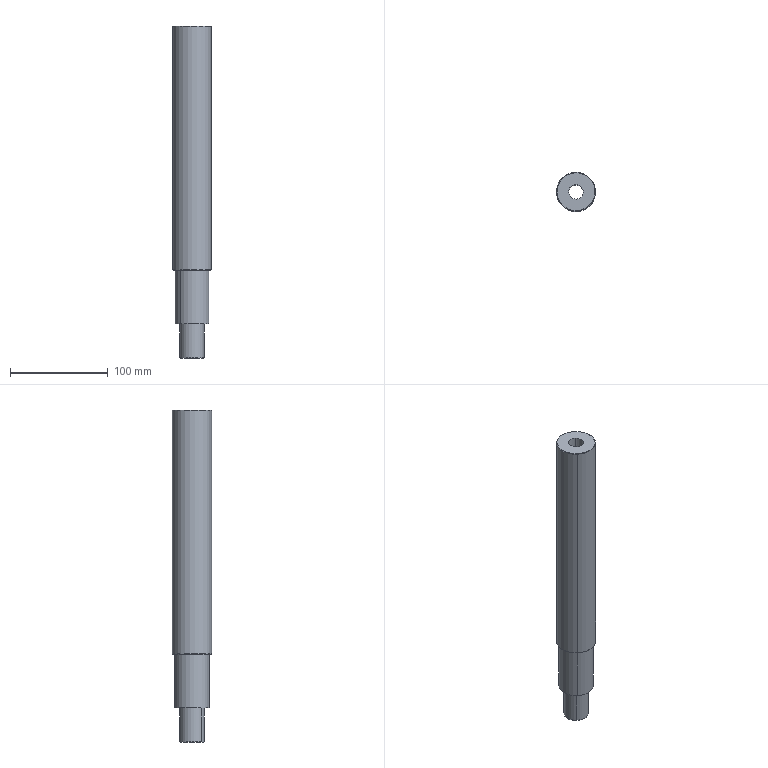Component | SolidWorks | 8TC-A17001-20-02HangingShaft-1 | 1 solid | 18 faces | box 40 x 40 x 340 mm | volume 324132 mm3 | cylinder 8 | cone 6 | plane 4 | commonest cylinder face diameters 40 x2 35 x2 25 x2 15 x2 | material #45
build123d program:
from build123d import *

# Parameters (mm, degrees)
CHAMFER1_SIZE = 0.5


with BuildPart() as part:
    # Sketch1 → Revolve1 (revolve)
    with BuildSketch(Plane(origin=(0, 0, 0), x_dir=(1, 0, 0), z_dir=(0, 1, 0)), mode=Mode.PRIVATE) as revolve1_sk:
        Polygon((0, 7.5), (0, 12.5), (35, 12.5), (35, 17.5), (90, 17.5), (90, 20), (340, 20), (340, 7.5), align=None)
    revolve(revolve1_sk.sketch.rotate(Axis((0, 0, 0), (1, 0, 0)), 180), axis=Axis((0, 0, 0), (1, 0, 0)))

    # Chamfer1
    chamfer1_edges = [part.edges().sort_by_distance(p)[0] for p in [
        (340, 0, -20),
        (90, 0, -20),
        (0, 0, -12.5),
    ]]
    chamfer(chamfer1_edges, length=CHAMFER1_SIZE)


solid = part.part

# Placed as in the assembly
solid = solid.moved(Location((733.029, 200.722, -47.5), (0, -90, 0)))
STEP:
#1=COLOUR_RGB('',0.7922,0.8196,0.9333);
#2=FILL_AREA_STYLE_COLOUR('',#1);
#3=FILL_AREA_STYLE('',(#2));
#4=SURFACE_STYLE_FILL_AREA(#3);
#5=SURFACE_SIDE_STYLE('',(#4));
#6=SURFACE_STYLE_USAGE(.BOTH.,#5);
#7=PRESENTATION_STYLE_ASSIGNMENT((#6));
#8=CARTESIAN_POINT('',(28.356,7.322,11.516));
#9=VERTEX_POINT('',#8);
#10=CARTESIAN_POINT('',(29.362,8.482,11.516));
#11=VERTEX_POINT('',#10);
#12=CARTESIAN_POINT('',(28.859,7.902,11.516));
#13=DIRECTION('',(0.,0.,1.));
#14=DIRECTION('',(0.6551,0.7555,0.));
#15=AXIS2_PLACEMENT_3D('',#12,#13,#14);
#16=CIRCLE('',#15,0.7677);
#17=EDGE_CURVE('',#9,#11,#16,.T.);
#18=ORIENTED_EDGE('',*,*,#17,.F.);
#19=CARTESIAN_POINT('',(28.344,7.308,11.496));
#20=VERTEX_POINT('',#19);
#21=CARTESIAN_POINT('',(28.344,7.308,11.496));
#22=DIRECTION('',(-0.4632,-0.5342,-0.7071));
#23=VECTOR('',#22,39.37);
#24=LINE('',#21,#23);
#25=EDGE_CURVE('',#9,#20,#24,.T.);
#26=ORIENTED_EDGE('',*,*,#25,.T.);
#27=CARTESIAN_POINT('',(29.375,8.497,11.496));
#28=VERTEX_POINT('',#27);
#29=CARTESIAN_POINT('',(28.859,7.902,11.496));
#30=DIRECTION('',(-0.,-0.,-1.));
#31=DIRECTION('',(0.6551,0.7555,0.));
#32=AXIS2_PLACEMENT_3D('',#29,#30,#31);
#33=CIRCLE('',#32,0.7874);
#34=EDGE_CURVE('',#28,#20,#33,.T.);
#35=ORIENTED_EDGE('',*,*,#34,.F.);
#36=CARTESIAN_POINT('',(29.375,8.497,11.496));
#37=DIRECTION('',(0.4632,0.5342,-0.7071));
#38=VECTOR('',#37,39.37);
#39=LINE('',#36,#38);
#40=EDGE_CURVE('',#11,#28,#39,.T.);
#41=ORIENTED_EDGE('',*,*,#40,.F.);
#42=EDGE_LOOP('',(#18,#26,#35,#41));
#43=FACE_OUTER_BOUND('',#42,.T.);
#44=CARTESIAN_POINT('',(28.859,7.902,11.496));
#45=DIRECTION('',(-0.,-0.,-1.));
#46=DIRECTION('',(0.6551,0.7555,0.));
#47=AXIS2_PLACEMENT_3D('',#44,#45,#46);
#48=CONICAL_SURFACE('',#47,0.7874,0.7854);
#49=ADVANCED_FACE('',(#43),#48,.T.);
#50=CARTESIAN_POINT('',(29.169,8.259,-1.87));
#51=VERTEX_POINT('',#50);
#52=CARTESIAN_POINT('',(28.55,7.545,-1.87));
#53=VERTEX_POINT('',#52);
#54=CARTESIAN_POINT('',(28.859,7.902,-1.87));
#55=DIRECTION('',(-0.,-0.,-1.));
#56=DIRECTION('',(-0.6551,-0.7555,0.));
#57=AXIS2_PLACEMENT_3D('',#54,#55,#56);
#58=CIRCLE('',#57,0.4724);
#59=EDGE_CURVE('',#51,#53,#58,.T.);
#60=ORIENTED_EDGE('',*,*,#59,.F.);
#61=CARTESIAN_POINT('',(29.182,8.274,-1.85));
#62=VERTEX_POINT('',#61);
#63=CARTESIAN_POINT('',(29.169,8.259,-1.87));
#64=DIRECTION('',(0.4632,0.5342,0.7071));
#65=VECTOR('',#64,39.37);
#66=LINE('',#63,#65);
#67=EDGE_CURVE('',#51,#62,#66,.T.);
#68=ORIENTED_EDGE('',*,*,#67,.T.);
#69=CARTESIAN_POINT('',(28.537,7.531,-1.85));
#70=VERTEX_POINT('',#69);
#71=CARTESIAN_POINT('',(28.859,7.902,-1.85));
#72=DIRECTION('',(0.,0.,1.));
#73=DIRECTION('',(-0.6551,-0.7555,0.));
#74=AXIS2_PLACEMENT_3D('',#71,#72,#73);
#75=CIRCLE('',#74,0.4921);
#76=EDGE_CURVE('',#70,#62,#75,.T.);
#77=ORIENTED_EDGE('',*,*,#76,.F.);
#78=CARTESIAN_POINT('',(28.55,7.545,-1.87));
#79=DIRECTION('',(-0.4632,-0.5342,0.7071));
#80=VECTOR('',#79,39.37);
#81=LINE('',#78,#80);
#82=EDGE_CURVE('',#53,#70,#81,.T.);
#83=ORIENTED_EDGE('',*,*,#82,.F.);
#84=EDGE_LOOP('',(#60,#68,#77,#83));
#85=FACE_OUTER_BOUND('',#84,.T.);
#86=CARTESIAN_POINT('',(28.859,7.902,-1.87));
#87=DIRECTION('',(0.,0.,1.));
#88=DIRECTION('',(-0.6551,-0.7555,0.));
#89=AXIS2_PLACEMENT_3D('',#86,#87,#88);
#90=CONICAL_SURFACE('',#89,0.4724,0.7854);
#91=ADVANCED_FACE('',(#85),#90,.T.);
#92=CARTESIAN_POINT('',(29.362,8.482,1.673));
#93=VERTEX_POINT('',#92);
#94=CARTESIAN_POINT('',(28.356,7.322,1.673));
#95=VERTEX_POINT('',#94);
#96=CARTESIAN_POINT('',(28.859,7.902,1.673));
#97=DIRECTION('',(-0.,-0.,-1.));
#98=DIRECTION('',(-0.6551,-0.7555,0.));
#99=AXIS2_PLACEMENT_3D('',#96,#97,#98);
#100=CIRCLE('',#99,0.7677);
#101=EDGE_CURVE('',#93,#95,#100,.T.);
#102=ORIENTED_EDGE('',*,*,#101,.F.);
#103=CARTESIAN_POINT('',(29.375,8.497,1.693));
#104=VERTEX_POINT('',#103);
#105=CARTESIAN_POINT('',(29.362,8.482,1.673));
#106=DIRECTION('',(0.4632,0.5342,0.7071));
#107=VECTOR('',#106,39.37);
#108=LINE('',#105,#107);
#109=EDGE_CURVE('',#93,#104,#108,.T.);
#110=ORIENTED_EDGE('',*,*,#109,.T.);
#111=CARTESIAN_POINT('',(28.344,7.308,1.693));
#112=VERTEX_POINT('',#111);
#113=CARTESIAN_POINT('',(28.859,7.902,1.693));
#114=DIRECTION('',(0.,0.,1.));
#115=DIRECTION('',(-0.6551,-0.7555,0.));
#116=AXIS2_PLACEMENT_3D('',#113,#114,#115);
#117=CIRCLE('',#116,0.7874);
#118=EDGE_CURVE('',#112,#104,#117,.T.);
#119=ORIENTED_EDGE('',*,*,#118,.F.);
#120=CARTESIAN_POINT('',(28.356,7.322,1.673));
#121=DIRECTION('',(-0.4632,-0.5342,0.7071));
#122=VECTOR('',#121,39.37);
#123=LINE('',#120,#122);
#124=EDGE_CURVE('',#95,#112,#123,.T.);
#125=ORIENTED_EDGE('',*,*,#124,.F.);
#126=EDGE_LOOP('',(#102,#110,#119,#125));
#127=FACE_OUTER_BOUND('',#126,.T.);
#128=CARTESIAN_POINT('',(28.859,7.902,1.673));
#129=DIRECTION('',(0.,0.,1.));
#130=DIRECTION('',(-0.6551,-0.7555,0.));
#131=AXIS2_PLACEMENT_3D('',#128,#129,#130);
#132=CONICAL_SURFACE('',#131,0.7677,0.7854);
#133=ADVANCED_FACE('',(#127),#132,.T.);
#134=ORIENTED_EDGE('',*,*,#34,.T.);
#135=CARTESIAN_POINT('',(28.344,7.308,-1.87));
#136=DIRECTION('',(-0.,-0.,-1.));
#137=VECTOR('',#136,39.37);
#138=LINE('',#135,#137);
#139=EDGE_CURVE('',#20,#112,#138,.T.);
#140=ORIENTED_EDGE('',*,*,#139,.T.);
#141=ORIENTED_EDGE('',*,*,#118,.T.);
#142=CARTESIAN_POINT('',(29.375,8.497,-1.87));
#143=DIRECTION('',(-0.,-0.,-1.));
#144=VECTOR('',#143,39.37);
#145=LINE('',#142,#144);
#146=EDGE_CURVE('',#28,#104,#145,.T.);
#147=ORIENTED_EDGE('',*,*,#146,.F.);
#148=EDGE_LOOP('',(#134,#140,#141,#147));
#149=FACE_OUTER_BOUND('',#148,.T.);
#150=CARTESIAN_POINT('',(28.859,7.902,-1.87));
#151=DIRECTION('',(-0.,-0.,-1.));
#152=DIRECTION('',(0.6551,0.7555,0.));
#153=AXIS2_PLACEMENT_3D('',#150,#151,#152);
#154=CYLINDRICAL_SURFACE('',#153,0.7874);
#155=ADVANCED_FACE('',(#149),#154,.T.);
#156=CARTESIAN_POINT('',(29.311,8.423,1.673));
#157=VERTEX_POINT('',#156);
#158=CARTESIAN_POINT('',(28.408,7.382,1.673));
#159=VERTEX_POINT('',#158);
#160=CARTESIAN_POINT('',(28.859,7.902,1.673));
#161=DIRECTION('',(-0.,-0.,-1.));
#162=DIRECTION('',(0.6551,0.7555,0.));
#163=AXIS2_PLACEMENT_3D('',#160,#161,#162);
#164=CIRCLE('',#163,0.689);
#165=EDGE_CURVE('',#157,#159,#164,.T.);
#166=ORIENTED_EDGE('',*,*,#165,.T.);
#167=CARTESIAN_POINT('',(28.408,7.382,-0.4921));
#168=VERTEX_POINT('',#167);
#169=CARTESIAN_POINT('',(28.408,7.382,-1.87));
#170=DIRECTION('',(-0.,-0.,-1.));
#171=VECTOR('',#170,39.37);
#172=LINE('',#169,#171);
#173=EDGE_CURVE('',#159,#168,#172,.T.);
#174=ORIENTED_EDGE('',*,*,#173,.T.);
#175=CARTESIAN_POINT('',(29.311,8.423,-0.4921));
#176=VERTEX_POINT('',#175);
#177=CARTESIAN_POINT('',(28.859,7.902,-0.4921));
#178=DIRECTION('',(-0.,-0.,-1.));
#179=DIRECTION('',(0.6551,0.7555,0.));
#180=AXIS2_PLACEMENT_3D('',#177,#178,#179);
#181=CIRCLE('',#180,0.689);
#182=EDGE_CURVE('',#176,#168,#181,.T.);
#183=ORIENTED_EDGE('',*,*,#182,.F.);
#184=CARTESIAN_POINT('',(29.311,8.423,-1.87));
#185=DIRECTION('',(-0.,-0.,-1.));
#186=VECTOR('',#185,39.37);
#187=LINE('',#184,#186);
#188=EDGE_CURVE('',#157,#176,#187,.T.);
#189=ORIENTED_EDGE('',*,*,#188,.F.);
#190=EDGE_LOOP('',(#166,#174,#183,#189));
#191=FACE_OUTER_BOUND('',#190,.T.);
#192=CARTESIAN_POINT('',(28.859,7.902,-1.87));
#193=DIRECTION('',(-0.,-0.,-1.));
#194=DIRECTION('',(0.6551,0.7555,0.));
#195=AXIS2_PLACEMENT_3D('',#192,#193,#194);
#196=CYLINDRICAL_SURFACE('',#195,0.689);
#197=ADVANCED_FACE('',(#191),#196,.T.);
#198=CARTESIAN_POINT('',(29.182,8.274,-0.4921));
#199=VERTEX_POINT('',#198);
#200=CARTESIAN_POINT('',(28.537,7.531,-0.4921));
#201=VERTEX_POINT('',#200);
#202=CARTESIAN_POINT('',(28.859,7.902,-0.4921));
#203=DIRECTION('',(-0.,-0.,-1.));
#204=DIRECTION('',(0.6551,0.7555,0.));
#205=AXIS2_PLACEMENT_3D('',#202,#203,#204);
#206=CIRCLE('',#205,0.4921);
#207=EDGE_CURVE('',#199,#201,#206,.T.);
#208=ORIENTED_EDGE('',*,*,#207,.T.);
#209=CARTESIAN_POINT('',(28.537,7.531,-1.87));
#210=DIRECTION('',(-0.,-0.,-1.));
#211=VECTOR('',#210,39.37);
#212=LINE('',#209,#211);
#213=EDGE_CURVE('',#201,#70,#212,.T.);
#214=ORIENTED_EDGE('',*,*,#213,.T.);
#215=ORIENTED_EDGE('',*,*,#76,.T.);
#216=CARTESIAN_POINT('',(29.182,8.274,-1.87));
#217=DIRECTION('',(-0.,-0.,-1.));
#218=VECTOR('',#217,39.37);
#219=LINE('',#216,#218);
#220=EDGE_CURVE('',#199,#62,#219,.T.);
#221=ORIENTED_EDGE('',*,*,#220,.F.);
#222=EDGE_LOOP('',(#208,#214,#215,#221));
#223=FACE_OUTER_BOUND('',#222,.T.);
#224=CARTESIAN_POINT('',(28.859,7.902,-1.87));
#225=DIRECTION('',(-0.,-0.,-1.));
#226=DIRECTION('',(0.6551,0.7555,0.));
#227=AXIS2_PLACEMENT_3D('',#224,#225,#226);
#228=CYLINDRICAL_SURFACE('',#227,0.4921);
#229=ADVANCED_FACE('',(#223),#228,.T.);
#230=CARTESIAN_POINT('',(28.666,7.679,11.516));
#231=VERTEX_POINT('',#230);
#232=CARTESIAN_POINT('',(29.053,8.126,11.516));
#233=VERTEX_POINT('',#232);
#234=CARTESIAN_POINT('',(28.859,7.902,11.516));
#235=DIRECTION('',(-0.,-0.,-1.));
#236=DIRECTION('',(0.6551,0.7555,0.));
#237=AXIS2_PLACEMENT_3D('',#234,#235,#236);
#238=CIRCLE('',#237,0.2953);
#239=EDGE_CURVE('',#231,#233,#238,.T.);
#240=ORIENTED_EDGE('',*,*,#239,.F.);
#241=CARTESIAN_POINT('',(28.666,7.679,-1.87));
#242=VERTEX_POINT('',#241);
#243=CARTESIAN_POINT('',(28.666,7.679,-1.87));
#244=DIRECTION('',(-0.,-0.,-1.));
#245=VECTOR('',#244,39.37);
#246=LINE('',#243,#245);
#247=EDGE_CURVE('',#231,#242,#246,.T.);
#248=ORIENTED_EDGE('',*,*,#247,.T.);
#249=CARTESIAN_POINT('',(29.053,8.126,-1.87));
#250=VERTEX_POINT('',#249);
#251=CARTESIAN_POINT('',(28.859,7.902,-1.87));
#252=DIRECTION('',(-0.,-0.,-1.));
#253=DIRECTION('',(0.6551,0.7555,0.));
#254=AXIS2_PLACEMENT_3D('',#251,#252,#253);
#255=CIRCLE('',#254,0.2953);
#256=EDGE_CURVE('',#242,#250,#255,.T.);
#257=ORIENTED_EDGE('',*,*,#256,.T.);
#258=CARTESIAN_POINT('',(29.053,8.126,-1.87));
#259=DIRECTION('',(-0.,-0.,-1.));
#260=VECTOR('',#259,39.37);
#261=LINE('',#258,#260);
#262=EDGE_CURVE('',#233,#250,#261,.T.);
#263=ORIENTED_EDGE('',*,*,#262,.F.);
#264=EDGE_LOOP('',(#240,#248,#257,#263));
#265=FACE_OUTER_BOUND('',#264,.T.);
#266=CARTESIAN_POINT('',(28.859,7.902,-1.87));
#267=DIRECTION('',(-0.,-0.,-1.));
#268=DIRECTION('',(0.6551,0.7555,0.));
#269=AXIS2_PLACEMENT_3D('',#266,#267,#268);
#270=CYLINDRICAL_SURFACE('',#269,0.2953);
#271=ADVANCED_FACE('',(#265),#270,.F.);
#272=ORIENTED_EDGE('',*,*,#247,.F.);
#273=CARTESIAN_POINT('',(28.859,7.902,11.516));
#274=DIRECTION('',(-0.,-0.,-1.));
#275=DIRECTION('',(0.6551,0.7555,0.));
#276=AXIS2_PLACEMENT_3D('',#273,#274,#275);
#277=CIRCLE('',#276,0.2953);
#278=EDGE_CURVE('',#233,#231,#277,.T.);
#279=ORIENTED_EDGE('',*,*,#278,.F.);
#280=ORIENTED_EDGE('',*,*,#262,.T.);
#281=CARTESIAN_POINT('',(28.859,7.902,-1.87));
#282=DIRECTION('',(-0.,-0.,-1.));
#283=DIRECTION('',(0.6551,0.7555,0.));
#284=AXIS2_PLACEMENT_3D('',#281,#282,#283);
#285=CIRCLE('',#284,0.2953);
#286=EDGE_CURVE('',#250,#242,#285,.T.);
#287=ORIENTED_EDGE('',*,*,#286,.T.);
#288=EDGE_LOOP('',(#272,#279,#280,#287));
#289=FACE_OUTER_BOUND('',#288,.T.);
#290=CARTESIAN_POINT('',(28.859,7.902,-1.87));
#291=DIRECTION('',(-0.,-0.,-1.));
#292=DIRECTION('',(0.6551,0.7555,0.));
#293=AXIS2_PLACEMENT_3D('',#290,#291,#292);
#294=CYLINDRICAL_SURFACE('',#293,0.2953);
#295=ADVANCED_FACE('',(#289),#294,.F.);
#296=CARTESIAN_POINT('',(28.859,7.902,-1.87));
#297=DIRECTION('',(-0.,-0.,-1.));
#298=DIRECTION('',(-0.6551,-0.7555,0.));
#299=AXIS2_PLACEMENT_3D('',#296,#297,#298);
#300=CIRCLE('',#299,0.4724);
#301=EDGE_CURVE('',#53,#51,#300,.T.);
#302=ORIENTED_EDGE('',*,*,#301,.T.);
#303=ORIENTED_EDGE('',*,*,#59,.T.);
#304=EDGE_LOOP('',(#302,#303));
#305=FACE_OUTER_BOUND('',#304,.T.);
#306=ORIENTED_EDGE('',*,*,#286,.F.);
#307=ORIENTED_EDGE('',*,*,#256,.F.);
#308=EDGE_LOOP('',(#306,#307));
#309=FACE_BOUND('',#308,.T.);
#310=CARTESIAN_POINT('',(28.666,7.679,-1.87));
#311=DIRECTION('',(0.,0.,1.));
#312=DIRECTION('',(-0.6551,-0.7555,0.));
#313=AXIS2_PLACEMENT_3D('',#310,#311,#312);
#314=PLANE('',#313);
#315=ADVANCED_FACE('',(#305,#309),#314,.F.);
#316=ORIENTED_EDGE('',*,*,#213,.F.);
#317=CARTESIAN_POINT('',(28.859,7.902,-0.4921));
#318=DIRECTION('',(-0.,-0.,-1.));
#319=DIRECTION('',(0.6551,0.7555,0.));
#320=AXIS2_PLACEMENT_3D('',#317,#318,#319);
#321=CIRCLE('',#320,0.4921);
#322=EDGE_CURVE('',#201,#199,#321,.T.);
#323=ORIENTED_EDGE('',*,*,#322,.T.);
#324=ORIENTED_EDGE('',*,*,#220,.T.);
#325=CARTESIAN_POINT('',(28.859,7.902,-1.85));
#326=DIRECTION('',(0.,0.,1.));
#327=DIRECTION('',(-0.6551,-0.7555,0.));
#328=AXIS2_PLACEMENT_3D('',#325,#326,#327);
#329=CIRCLE('',#328,0.4921);
#330=EDGE_CURVE('',#62,#70,#329,.T.);
#331=ORIENTED_EDGE('',*,*,#330,.T.);
#332=EDGE_LOOP('',(#316,#323,#324,#331));
#333=FACE_OUTER_BOUND('',#332,.T.);
#334=CARTESIAN_POINT('',(28.859,7.902,-1.87));
#335=DIRECTION('',(-0.,-0.,-1.));
#336=DIRECTION('',(0.6551,0.7555,0.));
#337=AXIS2_PLACEMENT_3D('',#334,#335,#336);
#338=CYLINDRICAL_SURFACE('',#337,0.4921);
#339=ADVANCED_FACE('',(#333),#338,.T.);
#340=ORIENTED_EDGE('',*,*,#207,.F.);
#341=ORIENTED_EDGE('',*,*,#322,.F.);
#342=EDGE_LOOP('',(#340,#341));
#343=FACE_BOUND('',#342,.T.);
#344=ORIENTED_EDGE('',*,*,#182,.T.);
#345=CARTESIAN_POINT('',(28.859,7.902,-0.4921));
#346=DIRECTION('',(-0.,-0.,-1.));
#347=DIRECTION('',(0.6551,0.7555,0.));
#348=AXIS2_PLACEMENT_3D('',#345,#346,#347);
#349=CIRCLE('',#348,0.689);
#350=EDGE_CURVE('',#168,#176,#349,.T.);
#351=ORIENTED_EDGE('',*,*,#350,.T.);
#352=EDGE_LOOP('',(#344,#351));
#353=FACE_OUTER_BOUND('',#352,.T.);
#354=CARTESIAN_POINT('',(28.537,7.531,-0.4921));
#355=DIRECTION('',(0.,0.,1.));
#356=DIRECTION('',(-0.6551,-0.7555,0.));
#357=AXIS2_PLACEMENT_3D('',#354,#355,#356);
#358=PLANE('',#357);
#359=ADVANCED_FACE('',(#343,#353),#358,.F.);
#360=ORIENTED_EDGE('',*,*,#173,.F.);
#361=CARTESIAN_POINT('',(28.859,7.902,1.673));
#362=DIRECTION('',(-0.,-0.,-1.));
#363=DIRECTION('',(0.6551,0.7555,0.));
#364=AXIS2_PLACEMENT_3D('',#361,#362,#363);
#365=CIRCLE('',#364,0.689);
#366=EDGE_CURVE('',#159,#157,#365,.T.);
#367=ORIENTED_EDGE('',*,*,#366,.T.);
#368=ORIENTED_EDGE('',*,*,#188,.T.);
#369=ORIENTED_EDGE('',*,*,#350,.F.);
#370=EDGE_LOOP('',(#360,#367,#368,#369));
#371=FACE_OUTER_BOUND('',#370,.T.);
#372=CARTESIAN_POINT('',(28.859,7.902,-1.87));
#373=DIRECTION('',(-0.,-0.,-1.));
#374=DIRECTION('',(0.6551,0.7555,0.));
#375=AXIS2_PLACEMENT_3D('',#372,#373,#374);
#376=CYLINDRICAL_SURFACE('',#375,0.689);
#377=ADVANCED_FACE('',(#371),#376,.T.);
#378=CARTESIAN_POINT('',(28.859,7.902,1.673));
#379=DIRECTION('',(-0.,-0.,-1.));
#380=DIRECTION('',(-0.6551,-0.7555,0.));
#381=AXIS2_PLACEMENT_3D('',#378,#379,#380);
#382=CIRCLE('',#381,0.7677);
#383=EDGE_CURVE('',#95,#93,#382,.T.);
#384=ORIENTED_EDGE('',*,*,#383,.T.);
#385=ORIENTED_EDGE('',*,*,#101,.T.);
#386=EDGE_LOOP('',(#384,#385));
#387=FACE_OUTER_BOUND('',#386,.T.);
#388=ORIENTED_EDGE('',*,*,#165,.F.);
#389=ORIENTED_EDGE('',*,*,#366,.F.);
#390=EDGE_LOOP('',(#388,#389));
#391=FACE_BOUND('',#390,.T.);
#392=CARTESIAN_POINT('',(28.408,7.382,1.673));
#393=DIRECTION('',(0.,0.,1.));
#394=DIRECTION('',(-0.6551,-0.7555,0.));
#395=AXIS2_PLACEMENT_3D('',#392,#393,#394);
#396=PLANE('',#395);
#397=ADVANCED_FACE('',(#387,#391),#396,.F.);
#398=ORIENTED_EDGE('',*,*,#139,.F.);
#399=CARTESIAN_POINT('',(28.859,7.902,11.496));
#400=DIRECTION('',(-0.,-0.,-1.));
#401=DIRECTION('',(0.6551,0.7555,0.));
#402=AXIS2_PLACEMENT_3D('',#399,#400,#401);
#403=CIRCLE('',#402,0.7874);
#404=EDGE_CURVE('',#20,#28,#403,.T.);
#405=ORIENTED_EDGE('',*,*,#404,.T.);
#406=ORIENTED_EDGE('',*,*,#146,.T.);
#407=CARTESIAN_POINT('',(28.859,7.902,1.693));
#408=DIRECTION('',(0.,0.,1.));
#409=DIRECTION('',(-0.6551,-0.7555,0.));
#410=AXIS2_PLACEMENT_3D('',#407,#408,#409);
#411=CIRCLE('',#410,0.7874);
#412=EDGE_CURVE('',#104,#112,#411,.T.);
#413=ORIENTED_EDGE('',*,*,#412,.T.);
#414=EDGE_LOOP('',(#398,#405,#406,#413));
#415=FACE_OUTER_BOUND('',#414,.T.);
#416=CARTESIAN_POINT('',(28.859,7.902,-1.87));
#417=DIRECTION('',(-0.,-0.,-1.));
#418=DIRECTION('',(0.6551,0.7555,0.));
#419=AXIS2_PLACEMENT_3D('',#416,#417,#418);
#420=CYLINDRICAL_SURFACE('',#419,0.7874);
#421=ADVANCED_FACE('',(#415),#420,.T.);
#422=CARTESIAN_POINT('',(28.859,7.902,11.516));
#423=DIRECTION('',(0.,0.,1.));
#424=DIRECTION('',(0.6551,0.7555,0.));
#425=AXIS2_PLACEMENT_3D('',#422,#423,#424);
#426=CIRCLE('',#425,0.7677);
#427=EDGE_CURVE('',#11,#9,#426,.T.);
#428=ORIENTED_EDGE('',*,*,#427,.T.);
#429=ORIENTED_EDGE('',*,*,#17,.T.);
#430=EDGE_LOOP('',(#428,#429));
#431=FACE_OUTER_BOUND('',#430,.T.);
#432=ORIENTED_EDGE('',*,*,#278,.T.);
#433=ORIENTED_EDGE('',*,*,#239,.T.);
#434=EDGE_LOOP('',(#432,#433));
#435=FACE_BOUND('',#434,.T.);
#436=CARTESIAN_POINT('',(28.344,7.308,11.516));
#437=DIRECTION('',(-0.,-0.,-1.));
#438=DIRECTION('',(0.6551,0.7555,-0.));
#439=AXIS2_PLACEMENT_3D('',#436,#437,#438);
#440=PLANE('',#439);
#441=ADVANCED_FACE('',(#431,#435),#440,.F.);
#442=ORIENTED_EDGE('',*,*,#109,.F.);
#443=ORIENTED_EDGE('',*,*,#383,.F.);
#444=ORIENTED_EDGE('',*,*,#124,.T.);
#445=ORIENTED_EDGE('',*,*,#412,.F.);
#446=EDGE_LOOP('',(#442,#443,#444,#445));
#447=FACE_OUTER_BOUND('',#446,.T.);
#448=CARTESIAN_POINT('',(28.859,7.902,1.673));
#449=DIRECTION('',(0.,0.,1.));
#450=DIRECTION('',(-0.6551,-0.7555,0.));
#451=AXIS2_PLACEMENT_3D('',#448,#449,#450);
#452=CONICAL_SURFACE('',#451,0.7677,0.7854);
#453=ADVANCED_FACE('',(#447),#452,.T.);
#454=ORIENTED_EDGE('',*,*,#67,.F.);
#455=ORIENTED_EDGE('',*,*,#301,.F.);
#456=ORIENTED_EDGE('',*,*,#82,.T.);
#457=ORIENTED_EDGE('',*,*,#330,.F.);
#458=EDGE_LOOP('',(#454,#455,#456,#457));
#459=FACE_OUTER_BOUND('',#458,.T.);
#460=CARTESIAN_POINT('',(28.859,7.902,-1.87));
#461=DIRECTION('',(0.,0.,1.));
#462=DIRECTION('',(-0.6551,-0.7555,0.));
#463=AXIS2_PLACEMENT_3D('',#460,#461,#462);
#464=CONICAL_SURFACE('',#463,0.4724,0.7854);
#465=ADVANCED_FACE('',(#459),#464,.T.);
#466=ORIENTED_EDGE('',*,*,#25,.F.);
#467=ORIENTED_EDGE('',*,*,#427,.F.);
#468=ORIENTED_EDGE('',*,*,#40,.T.);
#469=ORIENTED_EDGE('',*,*,#404,.F.);
#470=EDGE_LOOP('',(#466,#467,#468,#469));
#471=FACE_OUTER_BOUND('',#470,.T.);
#472=CARTESIAN_POINT('',(28.859,7.902,11.496));
#473=DIRECTION('',(-0.,-0.,-1.));
#474=DIRECTION('',(0.6551,0.7555,0.));
#475=AXIS2_PLACEMENT_3D('',#472,#473,#474);
#476=CONICAL_SURFACE('',#475,0.7874,0.7854);
#477=ADVANCED_FACE('',(#471),#476,.T.);
#478=CLOSED_SHELL('',(#49,#91,#133,#155,#197,#229,#271,#295,#315,#339,#359,#377,#397,#421,#441,#453,#465,#477));
#479=MANIFOLD_SOLID_BREP('',#478);
#480=STYLED_ITEM('',(#7),#479);
#481=(LENGTH_UNIT()NAMED_UNIT(*)SI_UNIT($,.METRE.));
#482=LENGTH_MEASURE_WITH_UNIT(LENGTH_MEASURE(0.0254),#481);
#483=DIMENSIONAL_EXPONENTS(1.,0.,0.,0.,0.,0.,0.);
#484=(CONVERSION_BASED_UNIT('',#482)LENGTH_UNIT()NAMED_UNIT(#483));
#485=UNCERTAINTY_MEASURE_WITH_UNIT(LENGTH_MEASURE(0.00001),#484,'','');
#486=(NAMED_UNIT(*)PLANE_ANGLE_UNIT()SI_UNIT($,.RADIAN.));
#487=(NAMED_UNIT(*)SI_UNIT($,.STERADIAN.)SOLID_ANGLE_UNIT());
#488=(GEOMETRIC_REPRESENTATION_CONTEXT(3)GLOBAL_UNCERTAINTY_ASSIGNED_CONTEXT((#485))GLOBAL_UNIT_ASSIGNED_CONTEXT((#484,#486,#487))REPRESENTATION_CONTEXT('',''));
#489=MECHANICAL_DESIGN_GEOMETRIC_PRESENTATION_REPRESENTATION('',(#480),#488);
#490=CARTESIAN_POINT('',(0.,0.,0.));
#491=DIRECTION('',(0.,0.,1.));
#492=DIRECTION('',(1.,0.,0.));
#493=AXIS2_PLACEMENT_3D('',#490,#491,#492);
#494=(LENGTH_UNIT()NAMED_UNIT(*)SI_UNIT($,.METRE.));
#495=LENGTH_MEASURE_WITH_UNIT(LENGTH_MEASURE(0.0254),#494);
#496=DIMENSIONAL_EXPONENTS(1.,0.,0.,0.,0.,0.,0.);
#497=(CONVERSION_BASED_UNIT('',#495)LENGTH_UNIT()NAMED_UNIT(#496));
#498=UNCERTAINTY_MEASURE_WITH_UNIT(LENGTH_MEASURE(0.00001),#497,'','');
#499=(NAMED_UNIT(*)PLANE_ANGLE_UNIT()SI_UNIT($,.RADIAN.));
#500=(NAMED_UNIT(*)SI_UNIT($,.STERADIAN.)SOLID_ANGLE_UNIT());
#501=(GEOMETRIC_REPRESENTATION_CONTEXT(3)GLOBAL_UNCERTAINTY_ASSIGNED_CONTEXT((#498))GLOBAL_UNIT_ASSIGNED_CONTEXT((#497,#499,#500))REPRESENTATION_CONTEXT('',''));
#502=ADVANCED_BREP_SHAPE_REPRESENTATION('',(#479,#493),#501);
#503=PRESENTATION_LAYER_ASSIGNMENT('','',(#480));